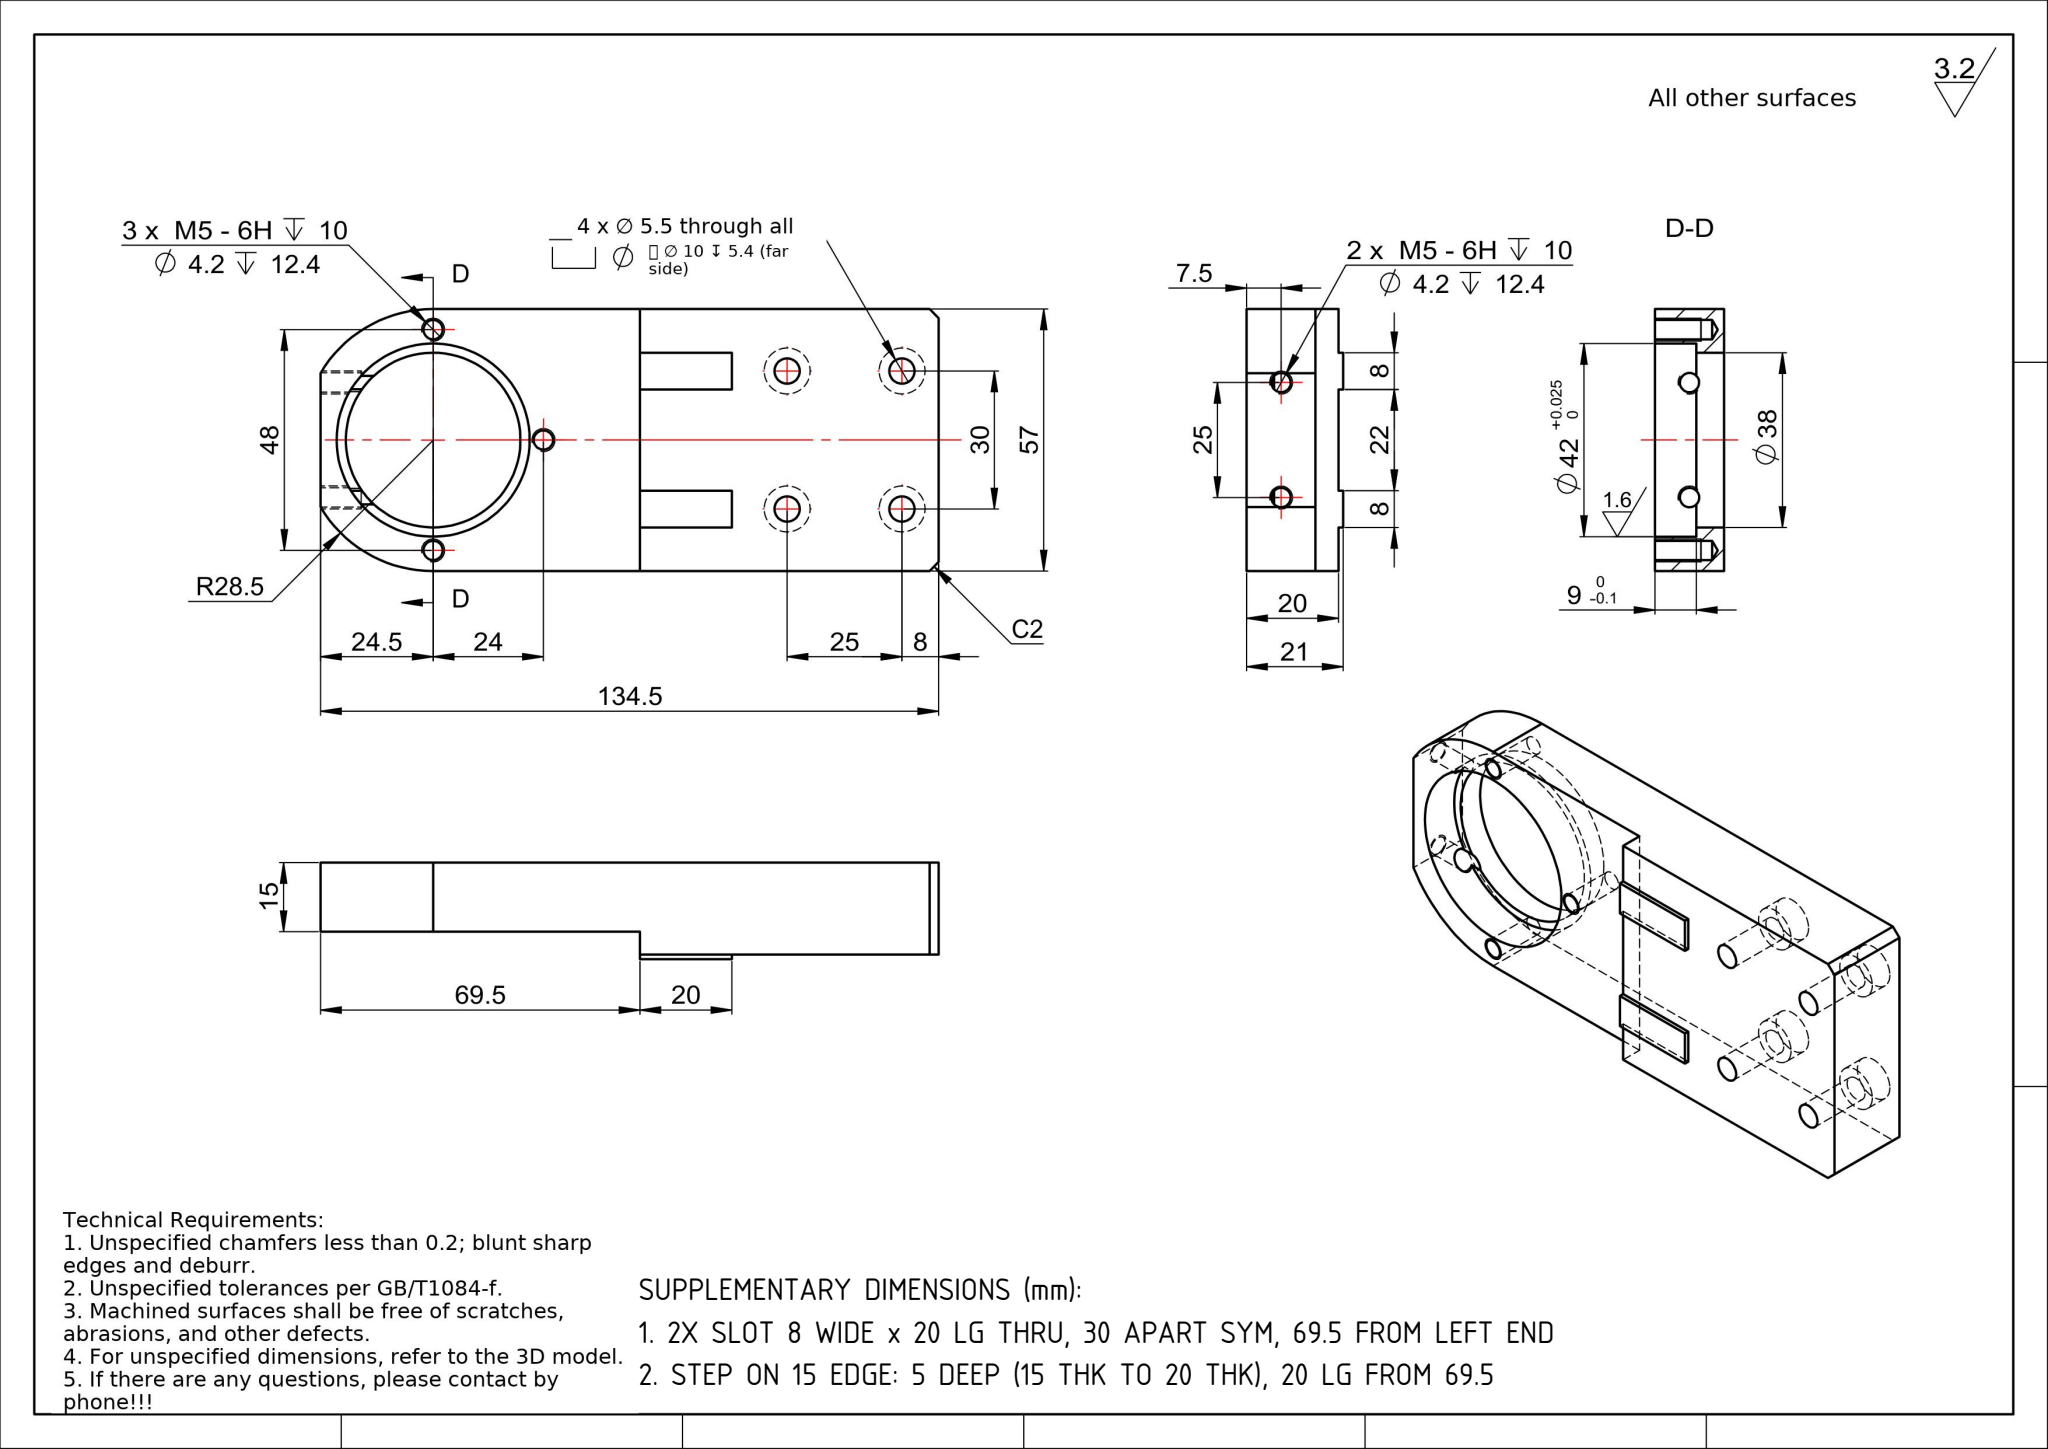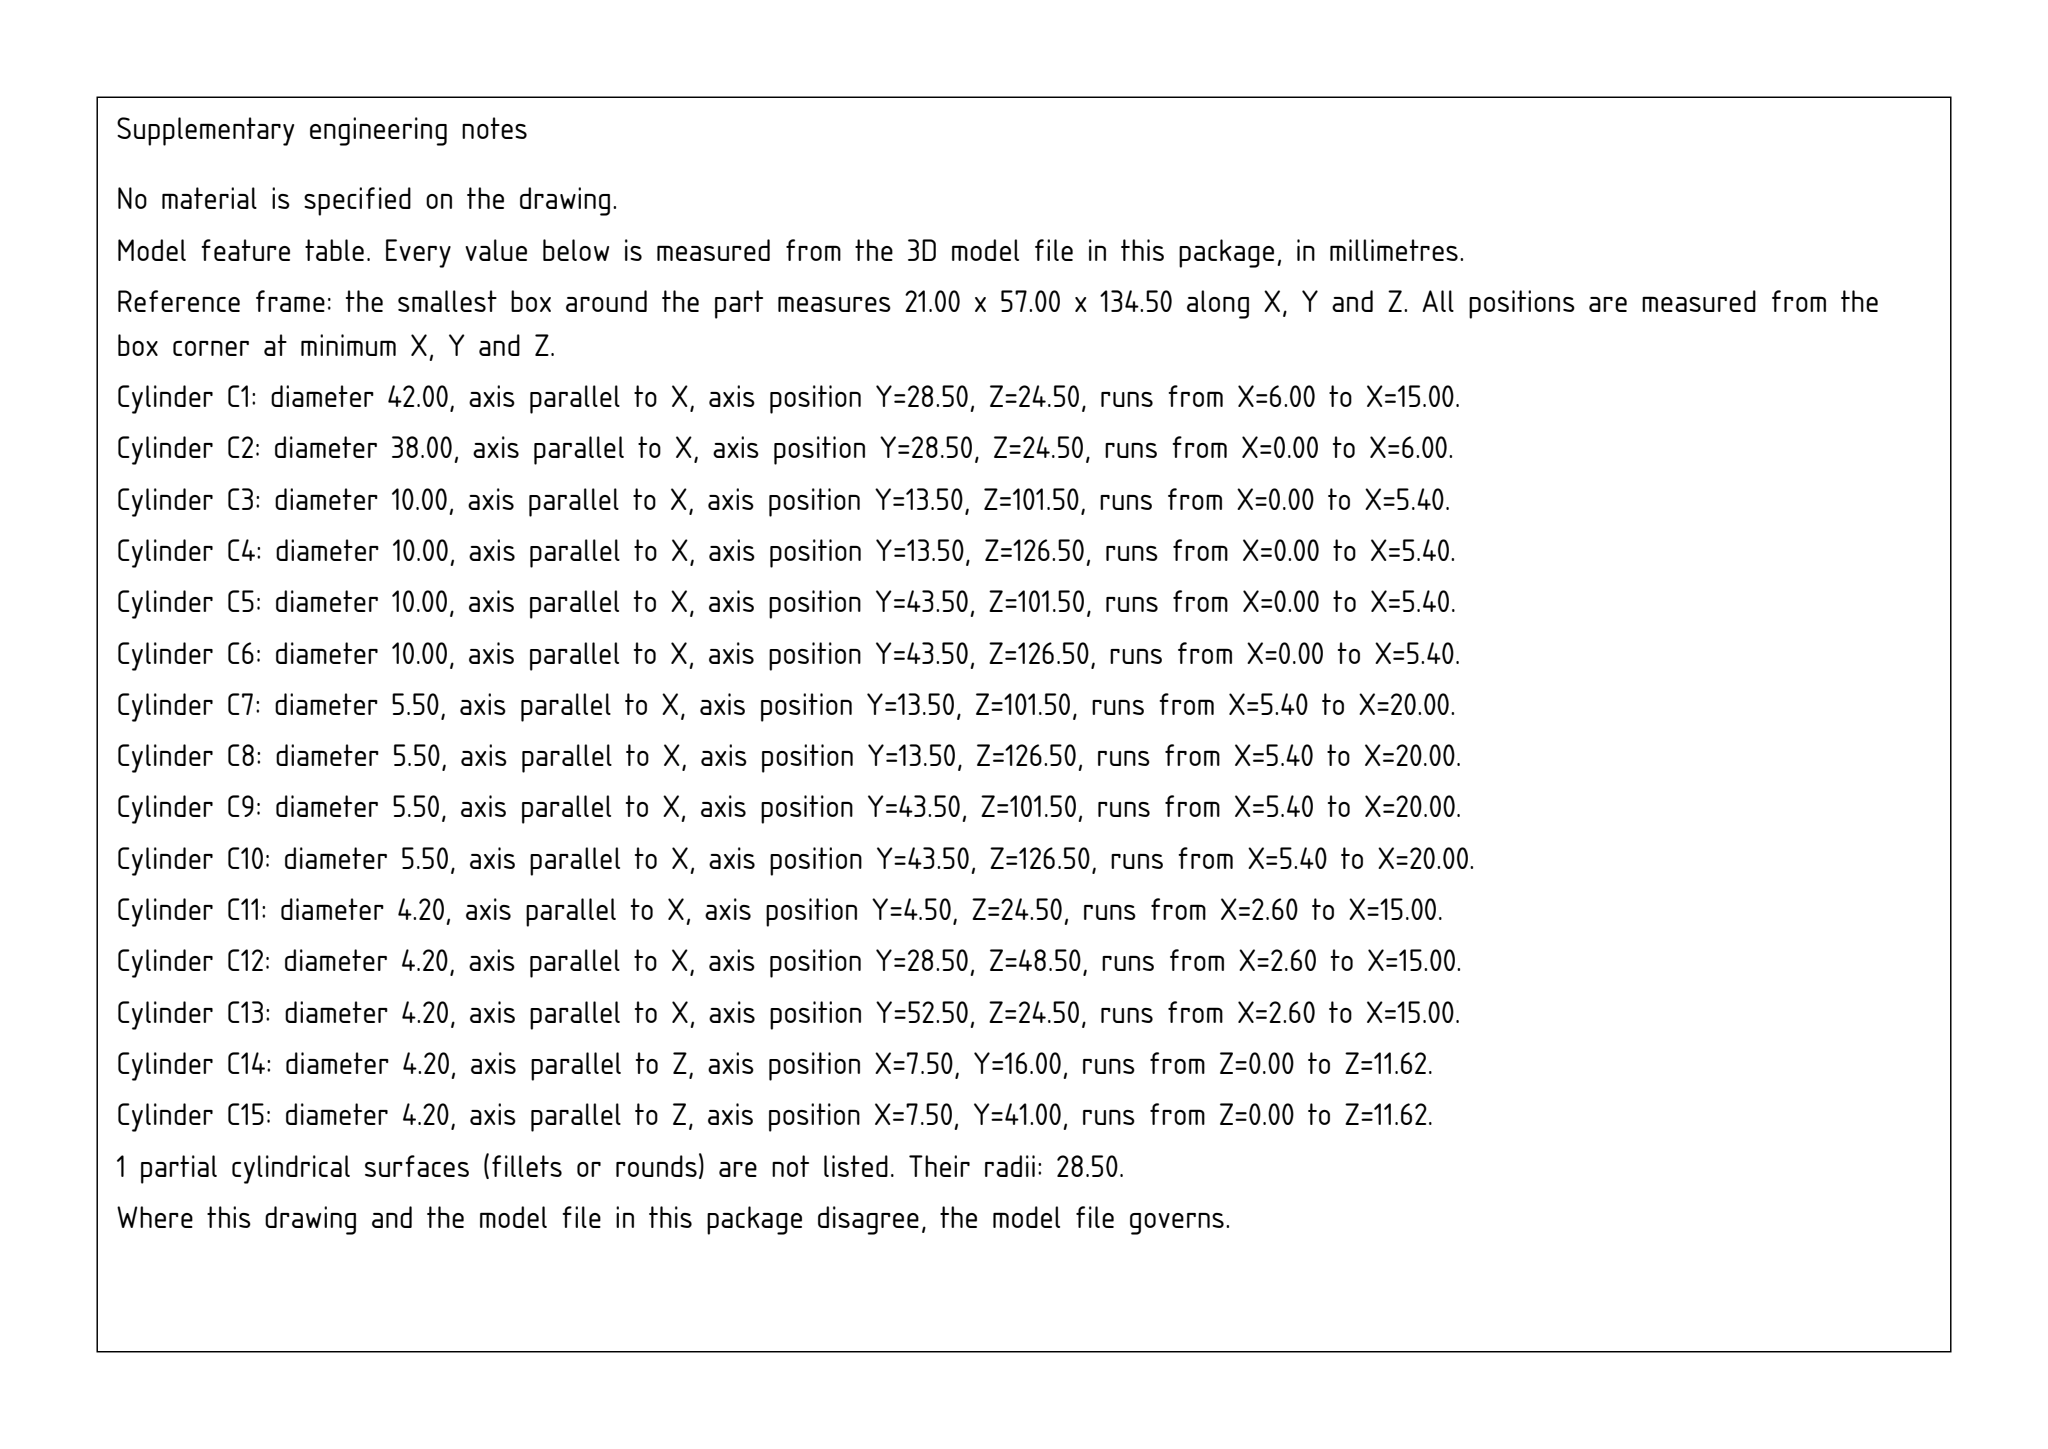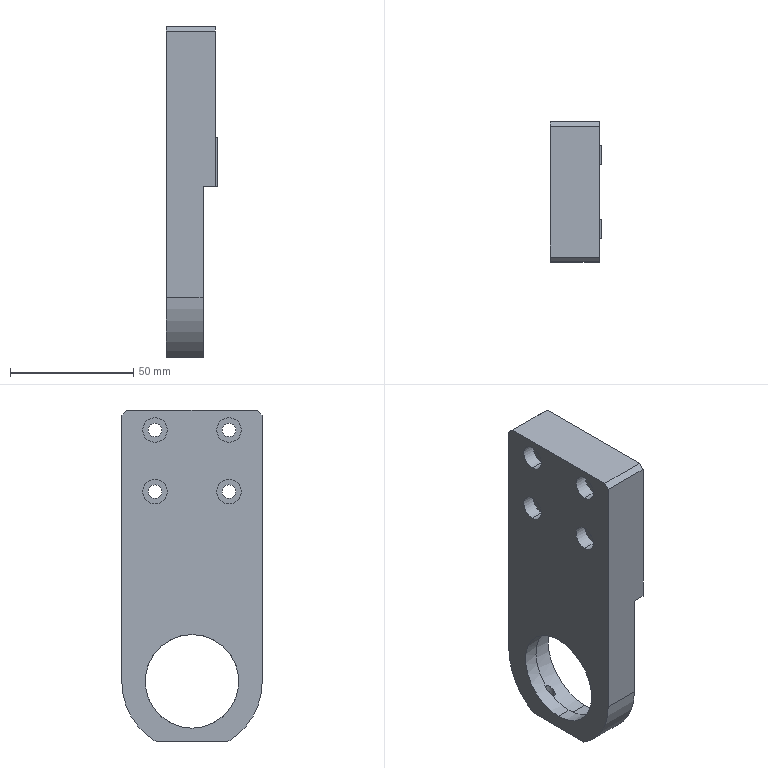Part | SolidWorks | mm | 1 solid | 62 faces | box 21 x 57 x 134.5 mm | volume 107662 mm3 | cylinder 32 | plane 24 | cone 6 | commonest cylinder face diameters 4.2 x10 10 x8 5.5 x8 38 x2 42 x2 57 x2
build123d program:
from build123d import *

# Parameters (mm, degrees)
BOSS_EXTRUDE1_DEPTH                             = 10
SKETCH2_R                                       = 19
CUT_EXTRUDE1_DEPTH                              = 127.183
SKETCH3_R                                       = 21
CUT_EXTRUDE2_DEPTH                              = 14
SKETCH4_W                                       = 80
SKETCH4_H                                       = 57
CUT_EXTRUDE3_DEPTH                              = 5
SKETCH17_W                                      = 20
SKETCH17_H                                      = 8
BOSS_EXTRUDE2_DEPTH                             = 1
SKETCH5_W                                       = 15
SKETCH5_H                                       = 50
CUT_EXTRUDE4_DEPTH                              = 4
M5_TAPPED_HOLE1_D                               = 4.2
M5_TAPPED_HOLE1_DEPTH                           = 12.4
M5_TAPPED_HOLE1_TIP                             = 1.262
M5_HEX_SOCKET_HEAD_CAP_SCREW_CBORE1_D           = 5.5
M5_HEX_SOCKET_HEAD_CAP_SCREW_CBORE1_CBORE_D     = 10
M5_HEX_SOCKET_HEAD_CAP_SCREW_CBORE1_CBORE_DEPTH = 5.4
M5_TAPPED_HOLE2_D                               = 4.2
M5_TAPPED_HOLE2_DEPTH                           = 12.4
M5_TAPPED_HOLE2_TIP                             = 1.262
CHAMFER1_SIZE                                   = 2


with BuildPart() as part:
    # Sketch1 → Boss-Extrude1 (new, symmetric)
    with BuildSketch(Plane(origin=(0, 0, 0), x_dir=(0, 0, -1), z_dir=(1, 0, 0))):
        with BuildLine():
            Line((0, -28.5), (-110, -28.5))
            Line((-110, -28.5), (-110, 28.5))
            Line((-110, 28.5), (0, 28.5))
            ThreePointArc((0, 28.5), (28.5, 0), (0, -28.5))
        make_face()
    extrude(amount=BOSS_EXTRUDE1_DEPTH, both=True)

    # Sketch2 → Cut-Extrude1 (cut, through all)
    with BuildSketch(Plane(origin=(10, 30, 0), x_dir=(0, 1, 0), z_dir=(-1, 0, 0))):
        with Locations(Location((-30, 0, 0), (0, 0, 270))):
            Circle(SKETCH2_R)
    extrude(amount=CUT_EXTRUDE1_DEPTH, mode=Mode.SUBTRACT)

    # Sketch3 → Cut-Extrude2 (cut)
    with BuildSketch(Plane(origin=(10, 0, 0), x_dir=(0, 0, -1), z_dir=(1, 0, 0))):
        Circle(SKETCH3_R)
    extrude(amount=-CUT_EXTRUDE2_DEPTH, mode=Mode.SUBTRACT)

    # Sketch4 → Cut-Extrude3 (cut)
    with BuildSketch(Plane(origin=(10, 0, 0), x_dir=(0, 0, -1), z_dir=(1, 0, 0))):
        with Locations((-5, 0)):
            Rectangle(SKETCH4_W, SKETCH4_H)
    extrude(amount=-CUT_EXTRUDE3_DEPTH, mode=Mode.SUBTRACT)

    # Sketch17 → Boss-Extrude2 (add)
    with BuildSketch(Plane(origin=(10, 0, 0), x_dir=(0, 0, -1), z_dir=(1, 0, 0))):
        with Locations((-55, 15)):
            Rectangle(SKETCH17_W, SKETCH17_H)
        with Locations((-55, -15)):
            Rectangle(SKETCH17_W, SKETCH17_H)
    extrude(amount=BOSS_EXTRUDE2_DEPTH)

    # Sketch5 → Cut-Extrude4 (cut)
    with BuildSketch(Plane(origin=(0, 0, -28.5), x_dir=(-1, 0, 0), z_dir=(0, 0, -1))):
        with Locations((2.5, 0)):
            Rectangle(SKETCH5_W, SKETCH5_H)
    extrude(amount=-CUT_EXTRUDE4_DEPTH, mode=Mode.SUBTRACT)

    # M5 Tapped Hole1
    with Locations(Plane(origin=(5, 0, 0), x_dir=(0, 0, -1), z_dir=(1, 0, 0))):
        with Locations((0, 24), (0, -24), (-24, 0)):
            Hole(M5_TAPPED_HOLE1_D / 2, depth=M5_TAPPED_HOLE1_DEPTH)
            with Locations((0, 0, -(M5_TAPPED_HOLE1_DEPTH + M5_TAPPED_HOLE1_TIP / 2))):  # 118° drill point
                Cone(0, M5_TAPPED_HOLE1_D / 2, M5_TAPPED_HOLE1_TIP, mode=Mode.SUBTRACT)

    # M5 Hex Socket Head Cap Screw CBORE1 (through all)
    with Locations(Plane.ZY.offset(10)):
        with Locations((77, 15), (102, -15), (77, -15), (102, 15)):
            CounterBoreHole(M5_HEX_SOCKET_HEAD_CAP_SCREW_CBORE1_D / 2, M5_HEX_SOCKET_HEAD_CAP_SCREW_CBORE1_CBORE_D / 2, M5_HEX_SOCKET_HEAD_CAP_SCREW_CBORE1_CBORE_DEPTH)

    # M5 Tapped Hole2
    with Locations(Plane(origin=(0, 0, -24.5), x_dir=(-1, 0, 0), z_dir=(0, 0, -1))):
        with Locations((2.5, 12.5), (2.5, -12.5)):
            Hole(M5_TAPPED_HOLE2_D / 2, depth=M5_TAPPED_HOLE2_DEPTH)
            with Locations((0, 0, -(M5_TAPPED_HOLE2_DEPTH + M5_TAPPED_HOLE2_TIP / 2))):  # 118° drill point
                Cone(0, M5_TAPPED_HOLE2_D / 2, M5_TAPPED_HOLE2_TIP, mode=Mode.SUBTRACT)

    # Chamfer1
    chamfer1_edges = [part.edges().sort_by_distance(p)[0] for p in [
        (0, -28.5, 110),
        (0, 28.5, 110),
    ]]
    chamfer(chamfer1_edges, length=CHAMFER1_SIZE)


solid = part.part